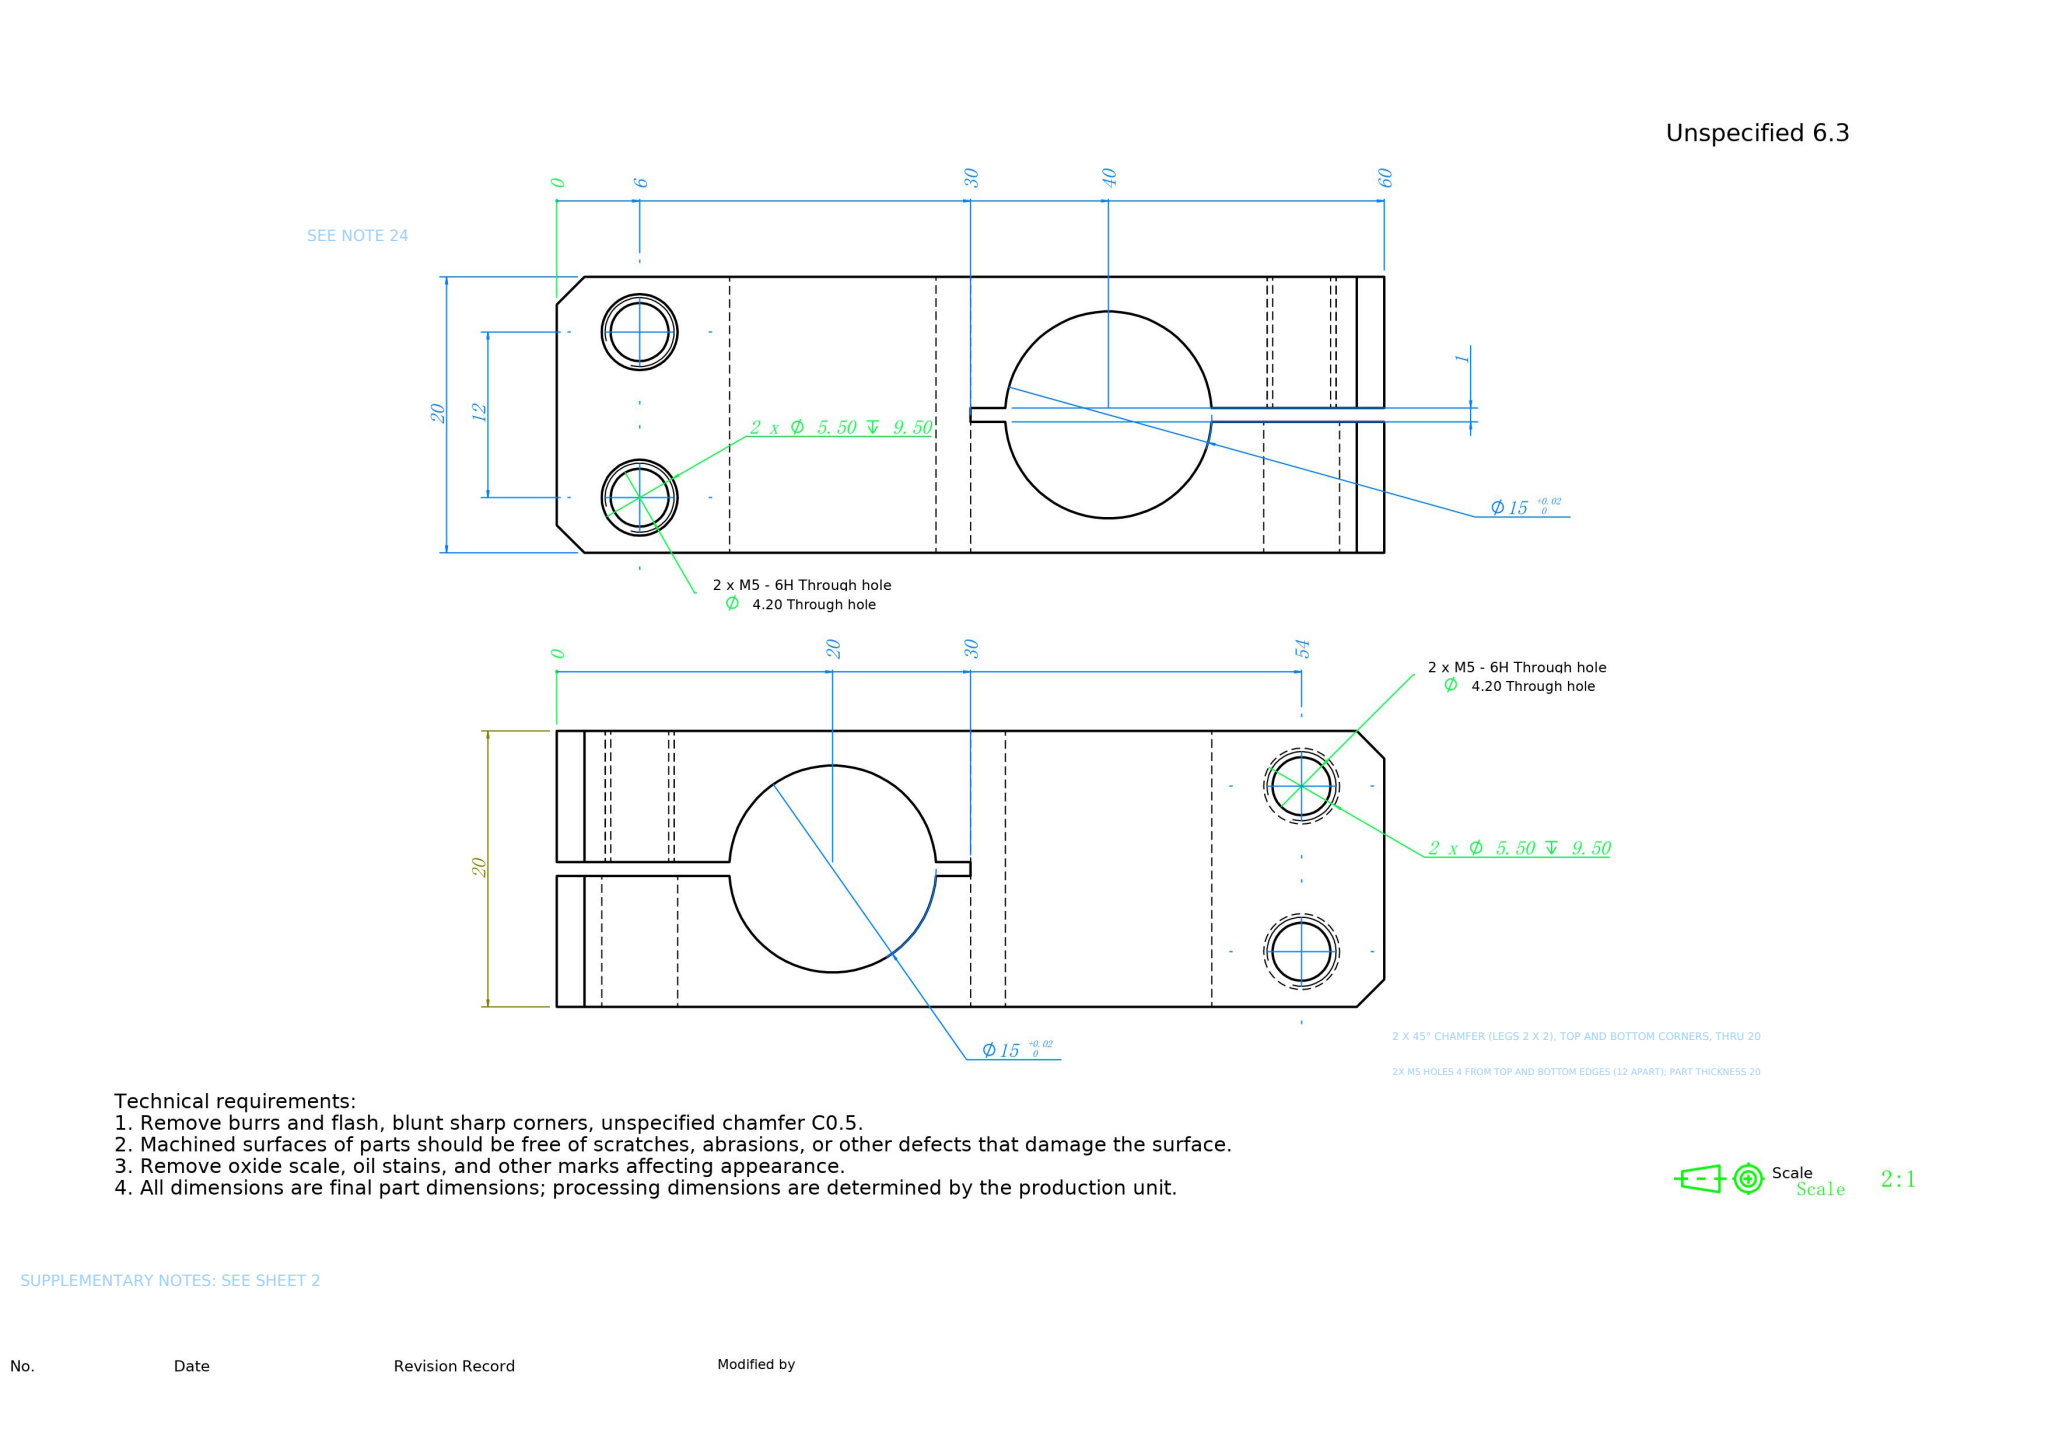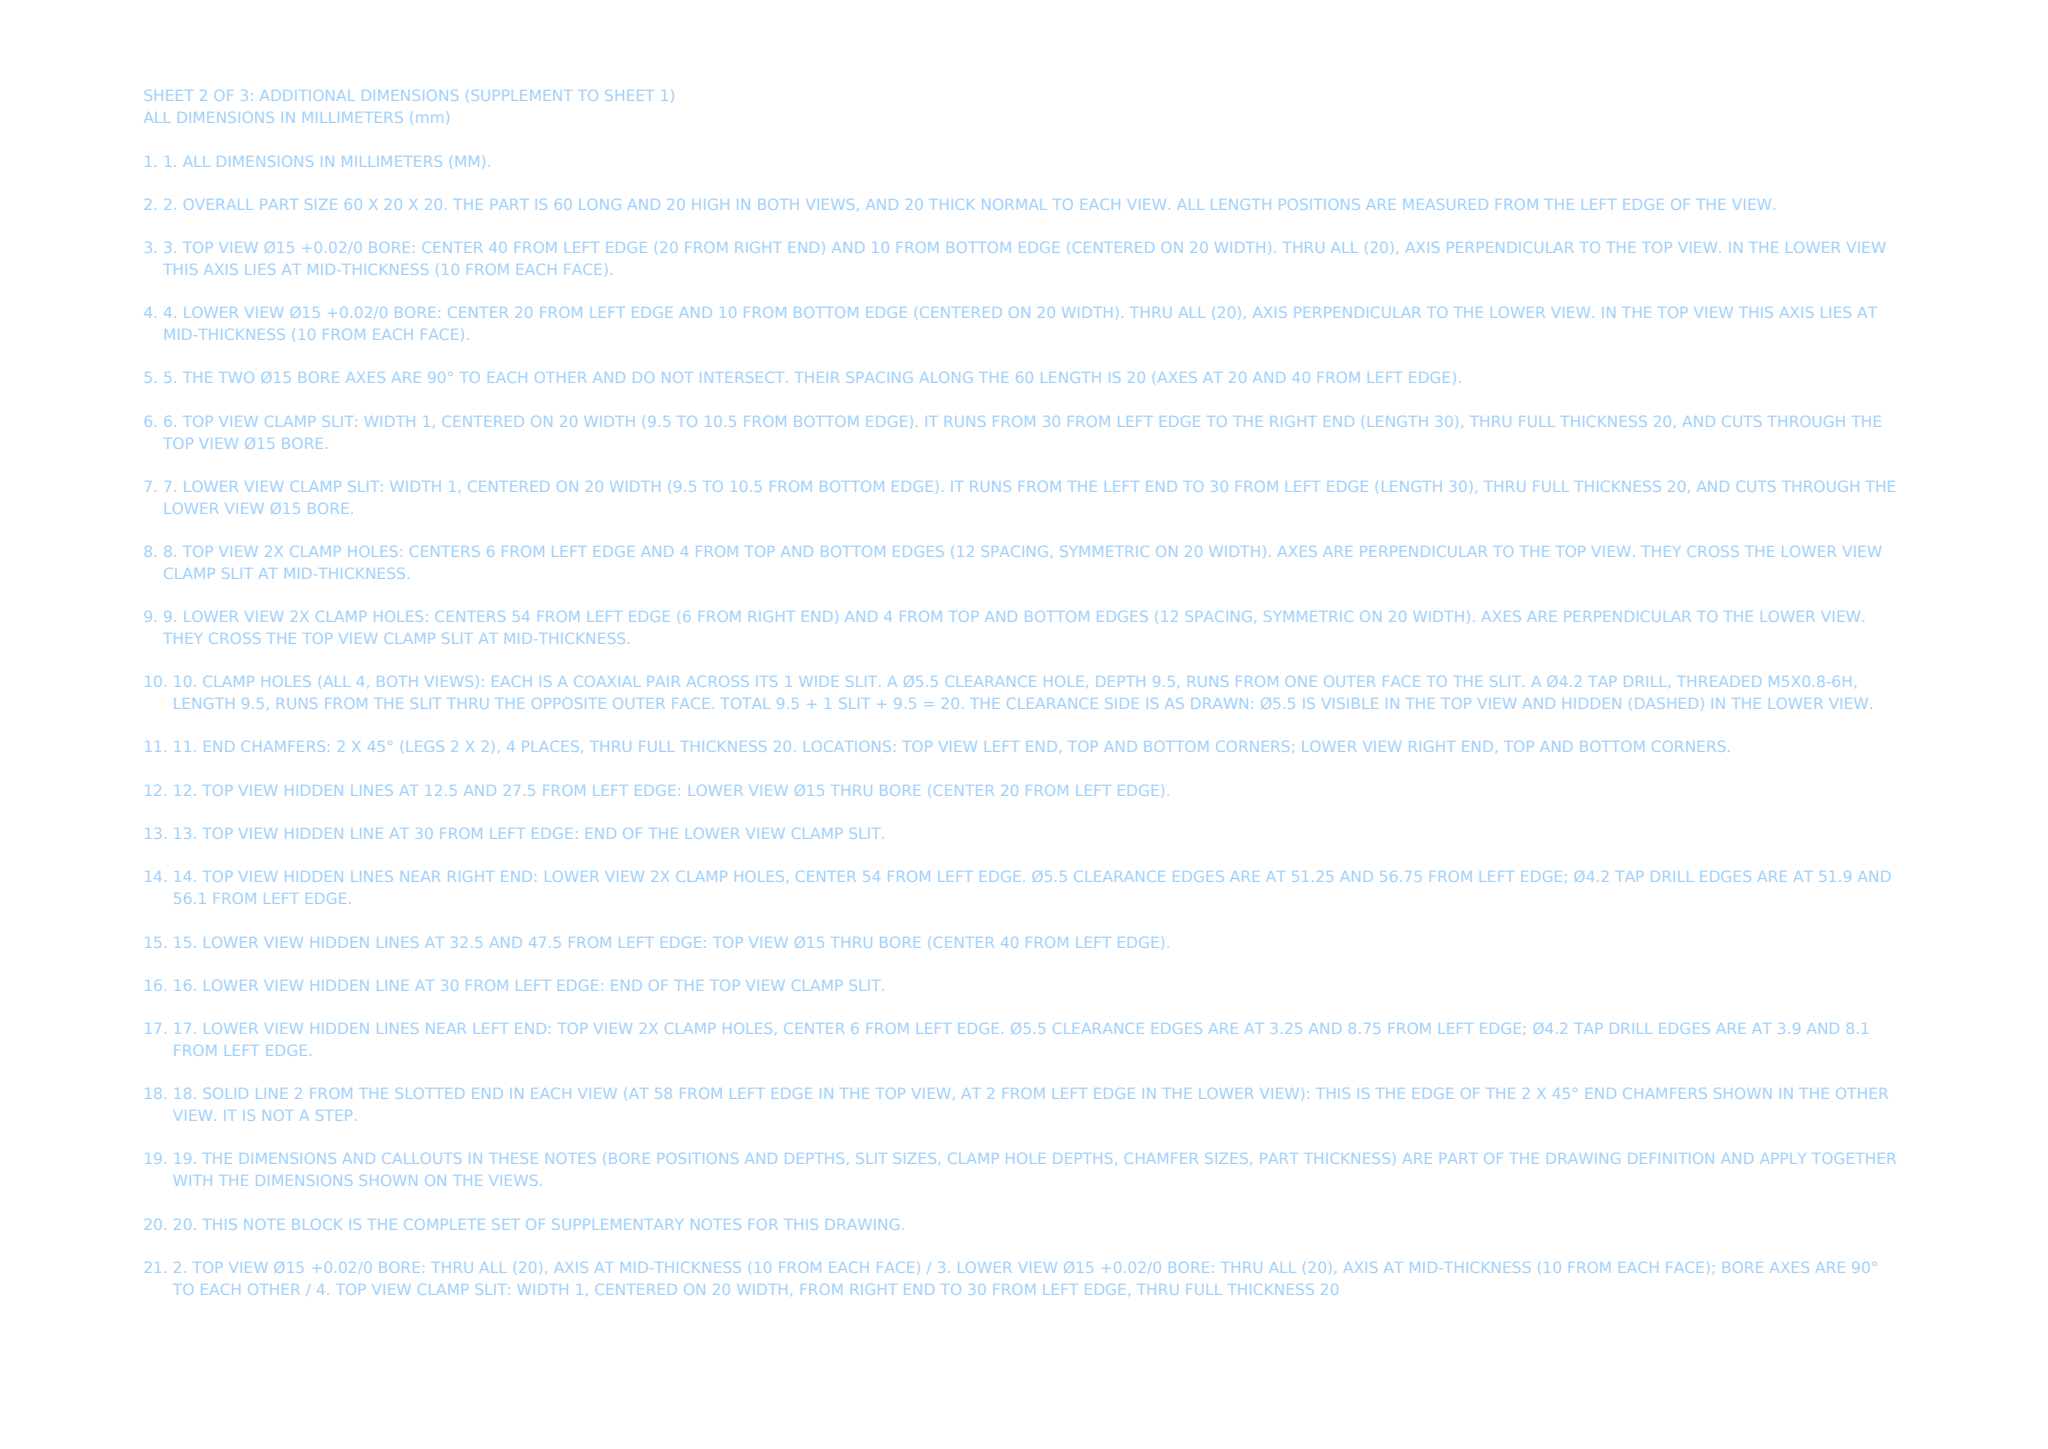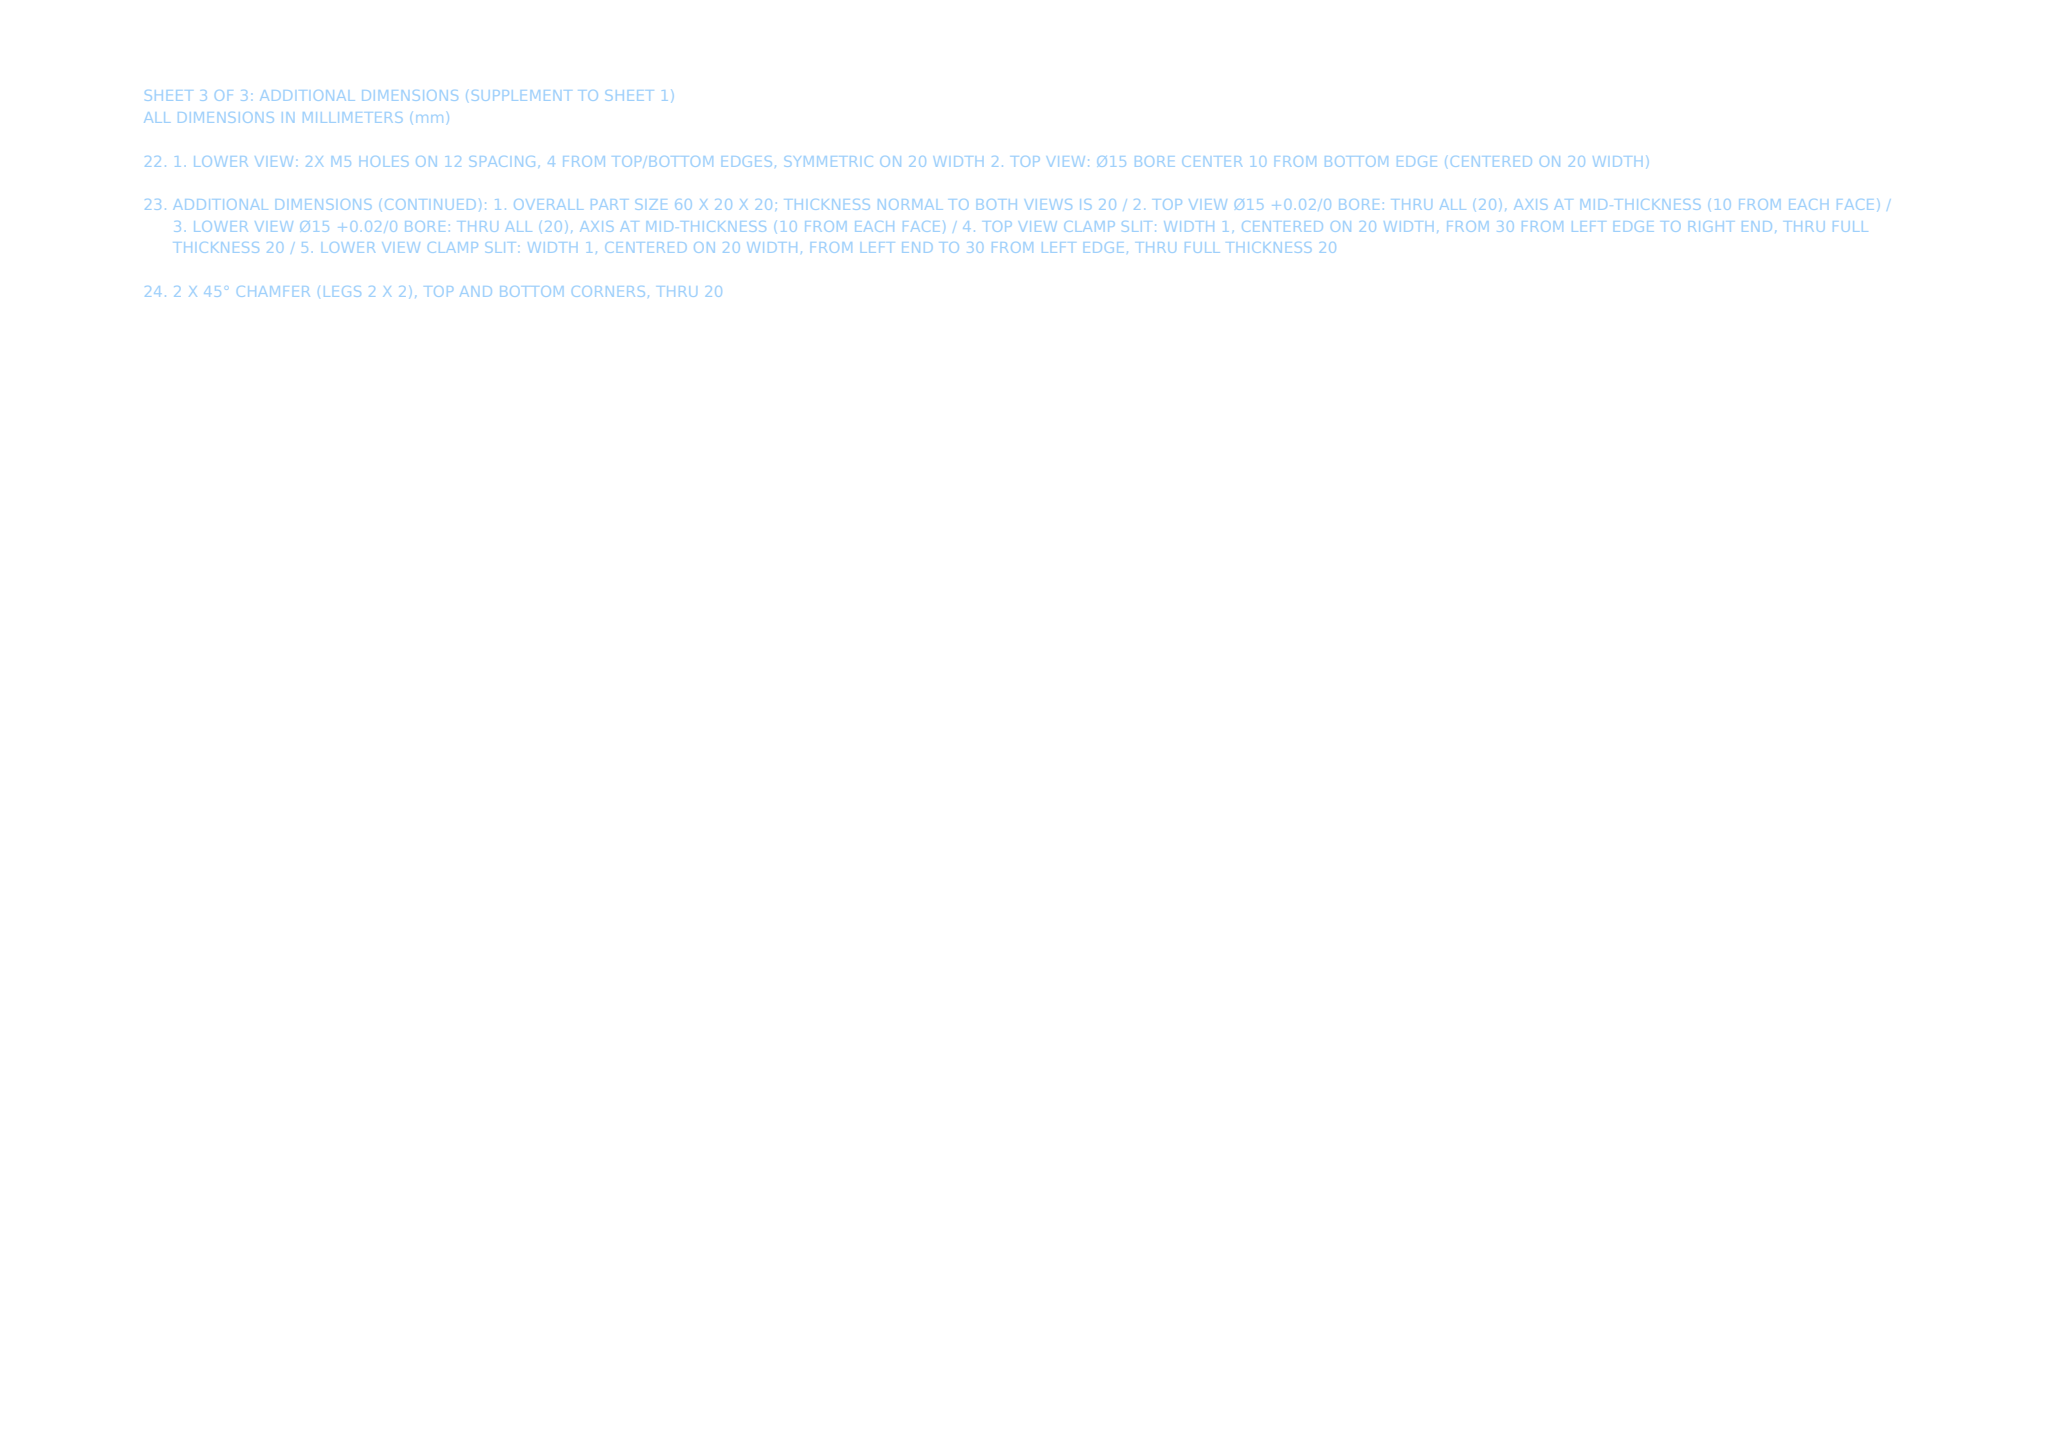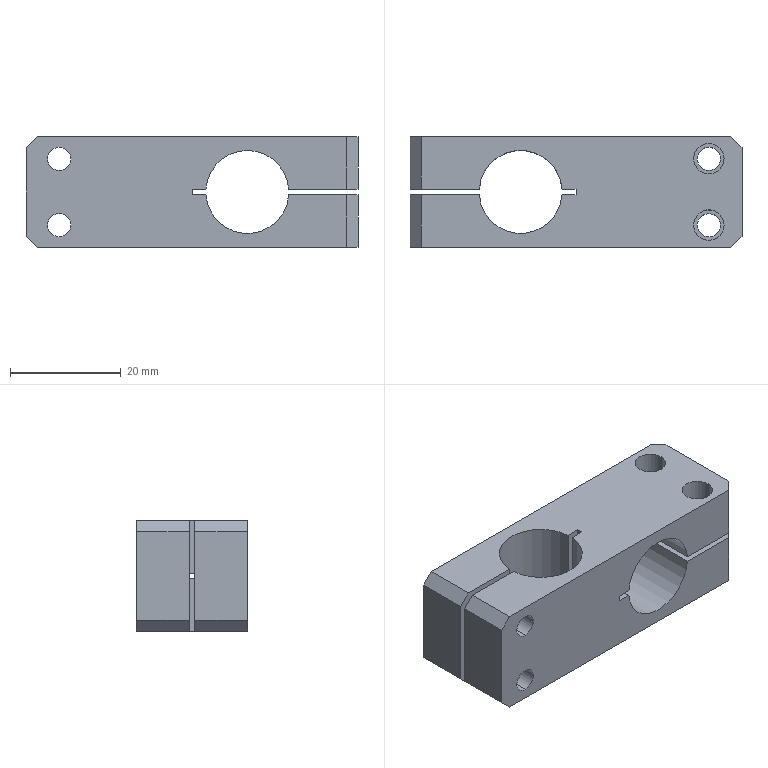Part | NX | mm | 1 solid | 49 faces | box 60 x 20 x 20 mm | volume 14750 mm3 | plane 28 | cylinder 21 | commonest cylinder face diameters 4.2 x8 5.5 x8 15 x5